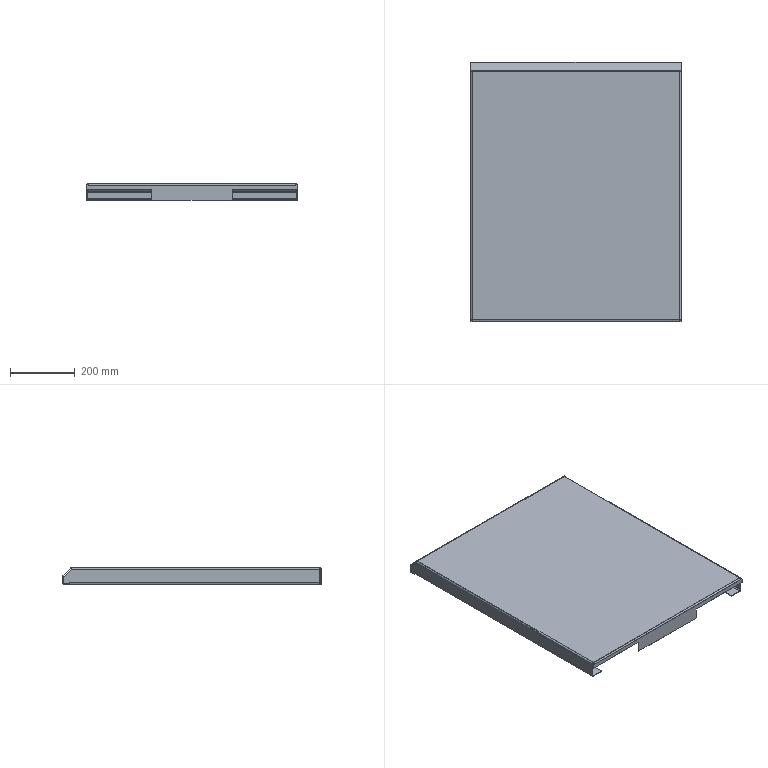Component | NX | SIDE_COVER_PLATE_FRONT_LEFT_2 | 1 solid | 72 faces | volume 1405358 mm3 | plane 54 | cylinder 18 | commonest cylinder face diameters 6 x10 10 x8